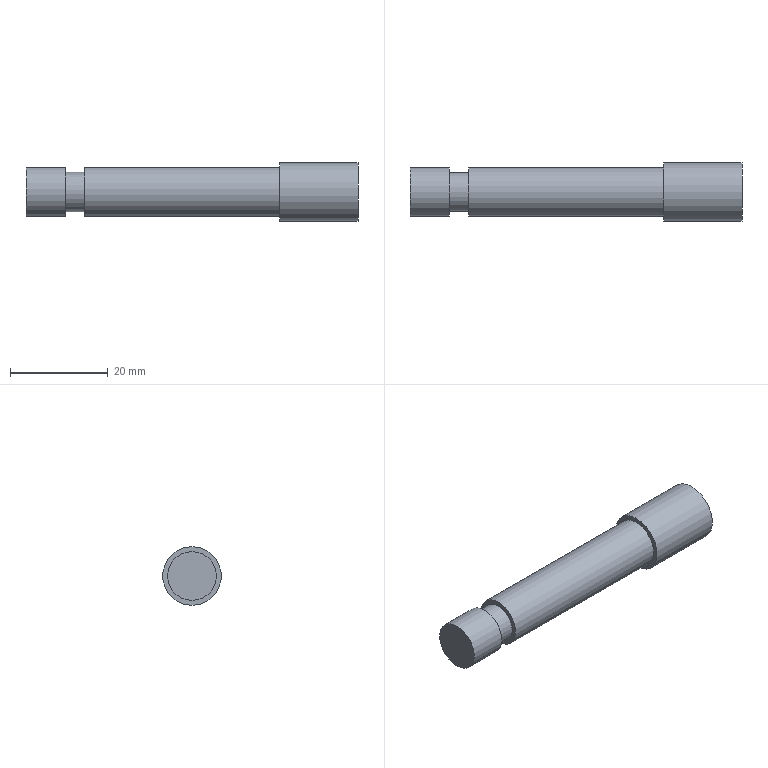Component | NX | THREADED_ROD | 1 solid | 9 faces | box 68 x 12 x 12 mm | volume 5781 mm3 | plane 5 | cylinder 4 | commonest cylinder face diameters 10 x2 8 x1 12 x1
STEP:
#1=CARTESIAN_POINT('',(0.,0.,0.));
#2=DIRECTION('',(0.,0.,1.));
#3=DIRECTION('',(1.,0.,0.));
#4=AXIS2_PLACEMENT_3D('',#1,#2,#3);
#5=CARTESIAN_POINT('',(780.009,-150.302,-1313.5));
#6=VERTEX_POINT('',#5);
#7=CARTESIAN_POINT('',(780.009,-150.302,-1307.5));
#8=DIRECTION('',(1.,0.,0.));
#9=DIRECTION('',(0.,0.,-1.));
#10=AXIS2_PLACEMENT_3D('',#7,#8,#9);
#11=CIRCLE('',#10,6.);
#12=CARTESIAN_POINT('',(780.009,-150.302,-1307.5));
#13=DIRECTION('',(1.,0.,0.));
#14=DIRECTION('',(0.,0.,-1.));
#15=AXIS2_PLACEMENT_3D('',#12,#13,#14);
#16=PLANE('',#15);
#17=CARTESIAN_POINT('',(0.,0.));
#18=DIRECTION('',(1.,0.));
#19=AXIS2_PLACEMENT_2D('',#17,#18);
#20=CIRCLE('',#19,6.);
#21=(GEOMETRIC_REPRESENTATION_CONTEXT(2)PARAMETRIC_REPRESENTATION_CONTEXT()REPRESENTATION_CONTEXT('',''));
#22=DEFINITIONAL_REPRESENTATION('',(#20),#21);
#23=PCURVE('',#16,#22);
#24=CARTESIAN_POINT('',(712.009,-150.302,-1307.5));
#25=DIRECTION('',(1.,0.,0.));
#26=DIRECTION('',(0.,0.,-1.));
#27=AXIS2_PLACEMENT_3D('',#24,#25,#26);
#28=CYLINDRICAL_SURFACE('',#27,6.);
#29=CARTESIAN_POINT('',(0.,68.));
#30=DIRECTION('',(1.,0.));
#31=VECTOR('',#30,1.);
#32=LINE('',#29,#31);
#33=(GEOMETRIC_REPRESENTATION_CONTEXT(2)PARAMETRIC_REPRESENTATION_CONTEXT()REPRESENTATION_CONTEXT('',''));
#34=DEFINITIONAL_REPRESENTATION('',(#32),#33);
#35=PCURVE('',#28,#34);
#36=SURFACE_CURVE('',#11,(#23,#35),.PCURVE_S1.);
#37=EDGE_CURVE('',#6,#6,#36,.T.);
#38=ORIENTED_EDGE('',*,*,#37,.T.);
#39=EDGE_LOOP('',(#38));
#40=FACE_BOUND('',#39,.T.);
#41=ADVANCED_FACE('',(#40),#16,.T.);
#42=CARTESIAN_POINT('',(712.009,-150.302,-1312.5));
#43=VERTEX_POINT('',#42);
#44=CARTESIAN_POINT('',(712.009,-150.302,-1307.5));
#45=DIRECTION('',(1.,0.,0.));
#46=DIRECTION('',(0.,0.,-1.));
#47=AXIS2_PLACEMENT_3D('',#44,#45,#46);
#48=CIRCLE('',#47,5.);
#49=CARTESIAN_POINT('',(712.009,-150.302,-1307.5));
#50=DIRECTION('',(1.,0.,0.));
#51=DIRECTION('',(0.,0.,-1.));
#52=AXIS2_PLACEMENT_3D('',#49,#50,#51);
#53=PLANE('',#52);
#54=CARTESIAN_POINT('',(0.,0.));
#55=DIRECTION('',(1.,0.));
#56=AXIS2_PLACEMENT_2D('',#54,#55);
#57=CIRCLE('',#56,5.);
#58=(GEOMETRIC_REPRESENTATION_CONTEXT(2)PARAMETRIC_REPRESENTATION_CONTEXT()REPRESENTATION_CONTEXT('',''));
#59=DEFINITIONAL_REPRESENTATION('',(#57),#58);
#60=PCURVE('',#53,#59);
#61=CARTESIAN_POINT('',(712.009,-150.302,-1307.5));
#62=DIRECTION('',(1.,0.,0.));
#63=DIRECTION('',(0.,0.,-1.));
#64=AXIS2_PLACEMENT_3D('',#61,#62,#63);
#65=CYLINDRICAL_SURFACE('',#64,5.);
#66=CARTESIAN_POINT('',(0.,0.));
#67=DIRECTION('',(1.,0.));
#68=VECTOR('',#67,1.);
#69=LINE('',#66,#68);
#70=(GEOMETRIC_REPRESENTATION_CONTEXT(2)PARAMETRIC_REPRESENTATION_CONTEXT()REPRESENTATION_CONTEXT('',''));
#71=DEFINITIONAL_REPRESENTATION('',(#69),#70);
#72=PCURVE('',#65,#71);
#73=SURFACE_CURVE('',#48,(#60,#72),.PCURVE_S1.);
#74=EDGE_CURVE('',#43,#43,#73,.T.);
#75=ORIENTED_EDGE('',*,*,#74,.F.);
#76=EDGE_LOOP('',(#75));
#77=FACE_BOUND('',#76,.T.);
#78=ADVANCED_FACE('',(#77),#53,.F.);
#79=ORIENTED_EDGE('',*,*,#74,.T.);
#80=CARTESIAN_POINT('',(720.009,-150.302,-1312.5));
#81=VERTEX_POINT('',#80);
#82=CARTESIAN_POINT('',(712.009,-150.302,-1312.5));
#83=CARTESIAN_POINT('',(720.009,-150.302,-1312.5));
#84=B_SPLINE_CURVE_WITH_KNOTS('',1,(#82,#83),.UNSPECIFIED.,.F.,.F.,(2,2),(0.,8.),.PIECEWISE_BEZIER_KNOTS.);
#85=CARTESIAN_POINT('',(6.283,0.));
#86=DIRECTION('',(0.,1.));
#87=VECTOR('',#86,1.);
#88=LINE('',#85,#87);
#89=(GEOMETRIC_REPRESENTATION_CONTEXT(2)PARAMETRIC_REPRESENTATION_CONTEXT()REPRESENTATION_CONTEXT('',''));
#90=DEFINITIONAL_REPRESENTATION('',(#88),#89);
#91=PCURVE('',#65,#90);
#92=CARTESIAN_POINT('',(0.,0.));
#93=DIRECTION('',(0.,1.));
#94=VECTOR('',#93,1.);
#95=LINE('',#92,#94);
#96=(GEOMETRIC_REPRESENTATION_CONTEXT(2)PARAMETRIC_REPRESENTATION_CONTEXT()REPRESENTATION_CONTEXT('',''));
#97=DEFINITIONAL_REPRESENTATION('',(#95),#96);
#98=PCURVE('',#65,#97);
#99=SEAM_CURVE('',#84,(#91,#98),.PCURVE_S1.);
#100=EDGE_CURVE('',#43,#81,#99,.T.);
#101=ORIENTED_EDGE('',*,*,#100,.T.);
#102=CARTESIAN_POINT('',(720.009,-150.302,-1307.5));
#103=DIRECTION('',(1.,0.,0.));
#104=DIRECTION('',(0.,0.,-1.));
#105=AXIS2_PLACEMENT_3D('',#102,#103,#104);
#106=CIRCLE('',#105,5.);
#107=CARTESIAN_POINT('',(0.,8.));
#108=DIRECTION('',(1.,0.));
#109=VECTOR('',#108,1.);
#110=LINE('',#107,#109);
#111=(GEOMETRIC_REPRESENTATION_CONTEXT(2)PARAMETRIC_REPRESENTATION_CONTEXT()REPRESENTATION_CONTEXT('',''));
#112=DEFINITIONAL_REPRESENTATION('',(#110),#111);
#113=PCURVE('',#65,#112);
#114=CARTESIAN_POINT('',(720.009,-150.302,-1303.5));
#115=DIRECTION('',(1.,0.,0.));
#116=DIRECTION('',(0.,0.,-1.));
#117=AXIS2_PLACEMENT_3D('',#114,#115,#116);
#118=PLANE('',#117);
#119=CARTESIAN_POINT('',(4.,0.));
#120=DIRECTION('',(1.,0.));
#121=AXIS2_PLACEMENT_2D('',#119,#120);
#122=CIRCLE('',#121,5.);
#123=(GEOMETRIC_REPRESENTATION_CONTEXT(2)PARAMETRIC_REPRESENTATION_CONTEXT()REPRESENTATION_CONTEXT('',''));
#124=DEFINITIONAL_REPRESENTATION('',(#122),#123);
#125=PCURVE('',#118,#124);
#126=SURFACE_CURVE('',#106,(#113,#125),.PCURVE_S1.);
#127=EDGE_CURVE('',#81,#81,#126,.T.);
#128=ORIENTED_EDGE('',*,*,#127,.F.);
#129=ORIENTED_EDGE('',*,*,#100,.F.);
#130=EDGE_LOOP('',(#79,#101,#128,#129));
#131=FACE_BOUND('',#130,.T.);
#132=ADVANCED_FACE('',(#131),#65,.T.);
#133=ORIENTED_EDGE('',*,*,#127,.T.);
#134=EDGE_LOOP('',(#133));
#135=FACE_BOUND('',#134,.T.);
#136=CARTESIAN_POINT('',(720.009,-150.302,-1311.5));
#137=VERTEX_POINT('',#136);
#138=CARTESIAN_POINT('',(720.009,-150.302,-1307.5));
#139=DIRECTION('',(1.,0.,0.));
#140=DIRECTION('',(0.,0.,-1.));
#141=AXIS2_PLACEMENT_3D('',#138,#139,#140);
#142=CIRCLE('',#141,4.);
#143=CARTESIAN_POINT('',(4.,0.));
#144=DIRECTION('',(1.,0.));
#145=AXIS2_PLACEMENT_2D('',#143,#144);
#146=CIRCLE('',#145,4.);
#147=(GEOMETRIC_REPRESENTATION_CONTEXT(2)PARAMETRIC_REPRESENTATION_CONTEXT()REPRESENTATION_CONTEXT('',''));
#148=DEFINITIONAL_REPRESENTATION('',(#146),#147);
#149=PCURVE('',#118,#148);
#150=CARTESIAN_POINT('',(712.009,-150.302,-1307.5));
#151=DIRECTION('',(1.,0.,0.));
#152=DIRECTION('',(0.,0.,-1.));
#153=AXIS2_PLACEMENT_3D('',#150,#151,#152);
#154=CYLINDRICAL_SURFACE('',#153,4.);
#155=CARTESIAN_POINT('',(0.,8.));
#156=DIRECTION('',(1.,0.));
#157=VECTOR('',#156,1.);
#158=LINE('',#155,#157);
#159=(GEOMETRIC_REPRESENTATION_CONTEXT(2)PARAMETRIC_REPRESENTATION_CONTEXT()REPRESENTATION_CONTEXT('',''));
#160=DEFINITIONAL_REPRESENTATION('',(#158),#159);
#161=PCURVE('',#154,#160);
#162=SURFACE_CURVE('',#142,(#149,#161),.PCURVE_S1.);
#163=EDGE_CURVE('',#137,#137,#162,.T.);
#164=ORIENTED_EDGE('',*,*,#163,.F.);
#165=EDGE_LOOP('',(#164));
#166=FACE_BOUND('',#165,.T.);
#167=ADVANCED_FACE('',(#135,#166),#118,.T.);
#168=ORIENTED_EDGE('',*,*,#163,.T.);
#169=CARTESIAN_POINT('',(724.009,-150.302,-1311.5));
#170=VERTEX_POINT('',#169);
#171=CARTESIAN_POINT('',(720.009,-150.302,-1311.5));
#172=CARTESIAN_POINT('',(724.009,-150.302,-1311.5));
#173=B_SPLINE_CURVE_WITH_KNOTS('',1,(#171,#172),.UNSPECIFIED.,.F.,.F.,(2,2),(8.,12.),.PIECEWISE_BEZIER_KNOTS.);
#174=CARTESIAN_POINT('',(6.283,0.));
#175=DIRECTION('',(0.,1.));
#176=VECTOR('',#175,1.);
#177=LINE('',#174,#176);
#178=(GEOMETRIC_REPRESENTATION_CONTEXT(2)PARAMETRIC_REPRESENTATION_CONTEXT()REPRESENTATION_CONTEXT('',''));
#179=DEFINITIONAL_REPRESENTATION('',(#177),#178);
#180=PCURVE('',#154,#179);
#181=CARTESIAN_POINT('',(0.,0.));
#182=DIRECTION('',(0.,1.));
#183=VECTOR('',#182,1.);
#184=LINE('',#181,#183);
#185=(GEOMETRIC_REPRESENTATION_CONTEXT(2)PARAMETRIC_REPRESENTATION_CONTEXT()REPRESENTATION_CONTEXT('',''));
#186=DEFINITIONAL_REPRESENTATION('',(#184),#185);
#187=PCURVE('',#154,#186);
#188=SEAM_CURVE('',#173,(#180,#187),.PCURVE_S1.);
#189=EDGE_CURVE('',#137,#170,#188,.T.);
#190=ORIENTED_EDGE('',*,*,#189,.T.);
#191=CARTESIAN_POINT('',(724.009,-150.302,-1307.5));
#192=DIRECTION('',(1.,0.,0.));
#193=DIRECTION('',(0.,0.,-1.));
#194=AXIS2_PLACEMENT_3D('',#191,#192,#193);
#195=CIRCLE('',#194,4.);
#196=CARTESIAN_POINT('',(0.,12.));
#197=DIRECTION('',(1.,0.));
#198=VECTOR('',#197,1.);
#199=LINE('',#196,#198);
#200=(GEOMETRIC_REPRESENTATION_CONTEXT(2)PARAMETRIC_REPRESENTATION_CONTEXT()REPRESENTATION_CONTEXT('',''));
#201=DEFINITIONAL_REPRESENTATION('',(#199),#200);
#202=PCURVE('',#154,#201);
#203=CARTESIAN_POINT('',(724.009,-150.302,-1302.5));
#204=DIRECTION('',(-1.,0.,0.));
#205=DIRECTION('',(0.,0.,1.));
#206=AXIS2_PLACEMENT_3D('',#203,#204,#205);
#207=PLANE('',#206);
#208=CARTESIAN_POINT('',(-9.,0.));
#209=CARTESIAN_POINT('',(-9.,6.928));
#210=CARTESIAN_POINT('',(-3.,3.464));
#211=CARTESIAN_POINT('',(3.,0.));
#212=CARTESIAN_POINT('',(-3.,-3.464));
#213=CARTESIAN_POINT('',(-9.,-6.928));
#214=CARTESIAN_POINT('',(-9.,0.));
#215=(BOUNDED_CURVE()B_SPLINE_CURVE(2,(#208,#209,#210,#211,#212,#213,#214),.UNSPECIFIED.,.T.,.F.)B_SPLINE_CURVE_WITH_KNOTS((1,2,2,2,2,1),(-2.094,0.,2.094,4.189,6.283,8.378),.UNSPECIFIED.)CURVE()GEOMETRIC_REPRESENTATION_ITEM()RATIONAL_B_SPLINE_CURVE((1.,0.5,1.,0.5,1.,0.5,1.))REPRESENTATION_ITEM(''));
#216=(GEOMETRIC_REPRESENTATION_CONTEXT(2)PARAMETRIC_REPRESENTATION_CONTEXT()REPRESENTATION_CONTEXT('',''));
#217=DEFINITIONAL_REPRESENTATION('',(#215),#216);
#218=PCURVE('',#207,#217);
#219=SURFACE_CURVE('',#195,(#202,#218),.PCURVE_S1.);
#220=EDGE_CURVE('',#170,#170,#219,.T.);
#221=ORIENTED_EDGE('',*,*,#220,.F.);
#222=ORIENTED_EDGE('',*,*,#189,.F.);
#223=EDGE_LOOP('',(#168,#190,#221,#222));
#224=FACE_BOUND('',#223,.T.);
#225=ADVANCED_FACE('',(#224),#154,.T.);
#226=ORIENTED_EDGE('',*,*,#220,.T.);
#227=EDGE_LOOP('',(#226));
#228=FACE_BOUND('',#227,.T.);
#229=CARTESIAN_POINT('',(724.009,-150.302,-1312.5));
#230=VERTEX_POINT('',#229);
#231=CARTESIAN_POINT('',(724.009,-150.302,-1307.5));
#232=DIRECTION('',(1.,0.,0.));
#233=DIRECTION('',(0.,0.,-1.));
#234=AXIS2_PLACEMENT_3D('',#231,#232,#233);
#235=CIRCLE('',#234,5.);
#236=CARTESIAN_POINT('',(-10.,0.));
#237=CARTESIAN_POINT('',(-10.,8.66));
#238=CARTESIAN_POINT('',(-2.5,4.33));
#239=CARTESIAN_POINT('',(5.,0.));
#240=CARTESIAN_POINT('',(-2.5,-4.33));
#241=CARTESIAN_POINT('',(-10.,-8.66));
#242=CARTESIAN_POINT('',(-10.,0.));
#243=(BOUNDED_CURVE()B_SPLINE_CURVE(2,(#236,#237,#238,#239,#240,#241,#242),.UNSPECIFIED.,.T.,.F.)B_SPLINE_CURVE_WITH_KNOTS((1,2,2,2,2,1),(-2.094,0.,2.094,4.189,6.283,8.378),.UNSPECIFIED.)CURVE()GEOMETRIC_REPRESENTATION_ITEM()RATIONAL_B_SPLINE_CURVE((1.,0.5,1.,0.5,1.,0.5,1.))REPRESENTATION_ITEM(''));
#244=(GEOMETRIC_REPRESENTATION_CONTEXT(2)PARAMETRIC_REPRESENTATION_CONTEXT()REPRESENTATION_CONTEXT('',''));
#245=DEFINITIONAL_REPRESENTATION('',(#243),#244);
#246=PCURVE('',#207,#245);
#247=CARTESIAN_POINT('',(712.009,-150.302,-1307.5));
#248=DIRECTION('',(1.,0.,0.));
#249=DIRECTION('',(0.,0.,-1.));
#250=AXIS2_PLACEMENT_3D('',#247,#248,#249);
#251=CYLINDRICAL_SURFACE('',#250,5.);
#252=CARTESIAN_POINT('',(0.,12.));
#253=DIRECTION('',(1.,0.));
#254=VECTOR('',#253,1.);
#255=LINE('',#252,#254);
#256=(GEOMETRIC_REPRESENTATION_CONTEXT(2)PARAMETRIC_REPRESENTATION_CONTEXT()REPRESENTATION_CONTEXT('',''));
#257=DEFINITIONAL_REPRESENTATION('',(#255),#256);
#258=PCURVE('',#251,#257);
#259=SURFACE_CURVE('',#235,(#246,#258),.PCURVE_S1.);
#260=EDGE_CURVE('',#230,#230,#259,.T.);
#261=ORIENTED_EDGE('',*,*,#260,.F.);
#262=EDGE_LOOP('',(#261));
#263=FACE_BOUND('',#262,.T.);
#264=ADVANCED_FACE('',(#228,#263),#207,.T.);
#265=ORIENTED_EDGE('',*,*,#260,.T.);
#266=CARTESIAN_POINT('',(764.009,-150.302,-1312.5));
#267=VERTEX_POINT('',#266);
#268=CARTESIAN_POINT('',(724.009,-150.302,-1312.5));
#269=CARTESIAN_POINT('',(764.009,-150.302,-1312.5));
#270=B_SPLINE_CURVE_WITH_KNOTS('',1,(#268,#269),.UNSPECIFIED.,.F.,.F.,(2,2),(12.,52.),.PIECEWISE_BEZIER_KNOTS.);
#271=CARTESIAN_POINT('',(6.283,0.));
#272=DIRECTION('',(0.,1.));
#273=VECTOR('',#272,1.);
#274=LINE('',#271,#273);
#275=(GEOMETRIC_REPRESENTATION_CONTEXT(2)PARAMETRIC_REPRESENTATION_CONTEXT()REPRESENTATION_CONTEXT('',''));
#276=DEFINITIONAL_REPRESENTATION('',(#274),#275);
#277=PCURVE('',#251,#276);
#278=CARTESIAN_POINT('',(0.,0.));
#279=DIRECTION('',(0.,1.));
#280=VECTOR('',#279,1.);
#281=LINE('',#278,#280);
#282=(GEOMETRIC_REPRESENTATION_CONTEXT(2)PARAMETRIC_REPRESENTATION_CONTEXT()REPRESENTATION_CONTEXT('',''));
#283=DEFINITIONAL_REPRESENTATION('',(#281),#282);
#284=PCURVE('',#251,#283);
#285=SEAM_CURVE('',#270,(#277,#284),.PCURVE_S1.);
#286=EDGE_CURVE('',#230,#267,#285,.T.);
#287=ORIENTED_EDGE('',*,*,#286,.T.);
#288=CARTESIAN_POINT('',(764.009,-150.302,-1307.5));
#289=DIRECTION('',(1.,0.,0.));
#290=DIRECTION('',(0.,0.,-1.));
#291=AXIS2_PLACEMENT_3D('',#288,#289,#290);
#292=CIRCLE('',#291,5.);
#293=CARTESIAN_POINT('',(0.,52.));
#294=DIRECTION('',(1.,0.));
#295=VECTOR('',#294,1.);
#296=LINE('',#293,#295);
#297=(GEOMETRIC_REPRESENTATION_CONTEXT(2)PARAMETRIC_REPRESENTATION_CONTEXT()REPRESENTATION_CONTEXT('',''));
#298=DEFINITIONAL_REPRESENTATION('',(#296),#297);
#299=PCURVE('',#251,#298);
#300=CARTESIAN_POINT('',(764.009,-150.302,-1301.5));
#301=DIRECTION('',(-1.,0.,0.));
#302=DIRECTION('',(0.,0.,1.));
#303=AXIS2_PLACEMENT_3D('',#300,#301,#302);
#304=PLANE('',#303);
#305=CARTESIAN_POINT('',(-11.,0.));
#306=CARTESIAN_POINT('',(-11.,8.66));
#307=CARTESIAN_POINT('',(-3.5,4.33));
#308=CARTESIAN_POINT('',(4.,0.));
#309=CARTESIAN_POINT('',(-3.5,-4.33));
#310=CARTESIAN_POINT('',(-11.,-8.66));
#311=CARTESIAN_POINT('',(-11.,0.));
#312=(BOUNDED_CURVE()B_SPLINE_CURVE(2,(#305,#306,#307,#308,#309,#310,#311),.UNSPECIFIED.,.T.,.F.)B_SPLINE_CURVE_WITH_KNOTS((1,2,2,2,2,1),(-2.094,0.,2.094,4.189,6.283,8.378),.UNSPECIFIED.)CURVE()GEOMETRIC_REPRESENTATION_ITEM()RATIONAL_B_SPLINE_CURVE((1.,0.5,1.,0.5,1.,0.5,1.))REPRESENTATION_ITEM(''));
#313=(GEOMETRIC_REPRESENTATION_CONTEXT(2)PARAMETRIC_REPRESENTATION_CONTEXT()REPRESENTATION_CONTEXT('',''));
#314=DEFINITIONAL_REPRESENTATION('',(#312),#313);
#315=PCURVE('',#304,#314);
#316=SURFACE_CURVE('',#292,(#299,#315),.PCURVE_S1.);
#317=EDGE_CURVE('',#267,#267,#316,.T.);
#318=ORIENTED_EDGE('',*,*,#317,.F.);
#319=ORIENTED_EDGE('',*,*,#286,.F.);
#320=EDGE_LOOP('',(#265,#287,#318,#319));
#321=FACE_BOUND('',#320,.T.);
#322=ADVANCED_FACE('',(#321),#251,.T.);
#323=ORIENTED_EDGE('',*,*,#317,.T.);
#324=EDGE_LOOP('',(#323));
#325=FACE_BOUND('',#324,.T.);
#326=CARTESIAN_POINT('',(764.009,-150.302,-1313.5));
#327=VERTEX_POINT('',#326);
#328=CARTESIAN_POINT('',(764.009,-150.302,-1307.5));
#329=DIRECTION('',(1.,0.,0.));
#330=DIRECTION('',(0.,0.,-1.));
#331=AXIS2_PLACEMENT_3D('',#328,#329,#330);
#332=CIRCLE('',#331,6.);
#333=CARTESIAN_POINT('',(-12.,0.));
#334=CARTESIAN_POINT('',(-12.,10.392));
#335=CARTESIAN_POINT('',(-3.,5.196));
#336=CARTESIAN_POINT('',(6.,0.));
#337=CARTESIAN_POINT('',(-3.,-5.196));
#338=CARTESIAN_POINT('',(-12.,-10.392));
#339=CARTESIAN_POINT('',(-12.,0.));
#340=(BOUNDED_CURVE()B_SPLINE_CURVE(2,(#333,#334,#335,#336,#337,#338,#339),.UNSPECIFIED.,.T.,.F.)B_SPLINE_CURVE_WITH_KNOTS((1,2,2,2,2,1),(-2.094,0.,2.094,4.189,6.283,8.378),.UNSPECIFIED.)CURVE()GEOMETRIC_REPRESENTATION_ITEM()RATIONAL_B_SPLINE_CURVE((1.,0.5,1.,0.5,1.,0.5,1.))REPRESENTATION_ITEM(''));
#341=(GEOMETRIC_REPRESENTATION_CONTEXT(2)PARAMETRIC_REPRESENTATION_CONTEXT()REPRESENTATION_CONTEXT('',''));
#342=DEFINITIONAL_REPRESENTATION('',(#340),#341);
#343=PCURVE('',#304,#342);
#344=CARTESIAN_POINT('',(0.,52.));
#345=DIRECTION('',(1.,0.));
#346=VECTOR('',#345,1.);
#347=LINE('',#344,#346);
#348=(GEOMETRIC_REPRESENTATION_CONTEXT(2)PARAMETRIC_REPRESENTATION_CONTEXT()REPRESENTATION_CONTEXT('',''));
#349=DEFINITIONAL_REPRESENTATION('',(#347),#348);
#350=PCURVE('',#28,#349);
#351=SURFACE_CURVE('',#332,(#343,#350),.PCURVE_S1.);
#352=EDGE_CURVE('',#327,#327,#351,.T.);
#353=ORIENTED_EDGE('',*,*,#352,.F.);
#354=EDGE_LOOP('',(#353));
#355=FACE_BOUND('',#354,.T.);
#356=ADVANCED_FACE('',(#325,#355),#304,.T.);
#357=ORIENTED_EDGE('',*,*,#352,.T.);
#358=CARTESIAN_POINT('',(764.009,-150.302,-1313.5));
#359=CARTESIAN_POINT('',(780.009,-150.302,-1313.5));
#360=B_SPLINE_CURVE_WITH_KNOTS('',1,(#358,#359),.UNSPECIFIED.,.F.,.F.,(2,2),(52.,68.),.PIECEWISE_BEZIER_KNOTS.);
#361=CARTESIAN_POINT('',(6.283,0.));
#362=DIRECTION('',(0.,1.));
#363=VECTOR('',#362,1.);
#364=LINE('',#361,#363);
#365=(GEOMETRIC_REPRESENTATION_CONTEXT(2)PARAMETRIC_REPRESENTATION_CONTEXT()REPRESENTATION_CONTEXT('',''));
#366=DEFINITIONAL_REPRESENTATION('',(#364),#365);
#367=PCURVE('',#28,#366);
#368=CARTESIAN_POINT('',(0.,0.));
#369=DIRECTION('',(0.,1.));
#370=VECTOR('',#369,1.);
#371=LINE('',#368,#370);
#372=(GEOMETRIC_REPRESENTATION_CONTEXT(2)PARAMETRIC_REPRESENTATION_CONTEXT()REPRESENTATION_CONTEXT('',''));
#373=DEFINITIONAL_REPRESENTATION('',(#371),#372);
#374=PCURVE('',#28,#373);
#375=SEAM_CURVE('',#360,(#367,#374),.PCURVE_S1.);
#376=EDGE_CURVE('',#327,#6,#375,.T.);
#377=ORIENTED_EDGE('',*,*,#376,.T.);
#378=ORIENTED_EDGE('',*,*,#37,.F.);
#379=ORIENTED_EDGE('',*,*,#376,.F.);
#380=EDGE_LOOP('',(#357,#377,#378,#379));
#381=FACE_BOUND('',#380,.T.);
#382=ADVANCED_FACE('',(#381),#28,.T.);
#383=CLOSED_SHELL('',(#41,#78,#132,#167,#225,#264,#322,#356,#382));
#384=MANIFOLD_SOLID_BREP('',#383);
#385=(LENGTH_UNIT()NAMED_UNIT(*)SI_UNIT(.MILLI.,.METRE.));
#386=UNCERTAINTY_MEASURE_WITH_UNIT(LENGTH_MEASURE(0.00001),#385,'','');
#387=(NAMED_UNIT(*)PLANE_ANGLE_UNIT()SI_UNIT($,.RADIAN.));
#388=(NAMED_UNIT(*)SI_UNIT($,.STERADIAN.)SOLID_ANGLE_UNIT());
#389=(GEOMETRIC_REPRESENTATION_CONTEXT(3)GLOBAL_UNCERTAINTY_ASSIGNED_CONTEXT((#386))GLOBAL_UNIT_ASSIGNED_CONTEXT((#385,#387,#388))REPRESENTATION_CONTEXT('',''));
#390=ADVANCED_BREP_SHAPE_REPRESENTATION('',(#4,#384),#389);